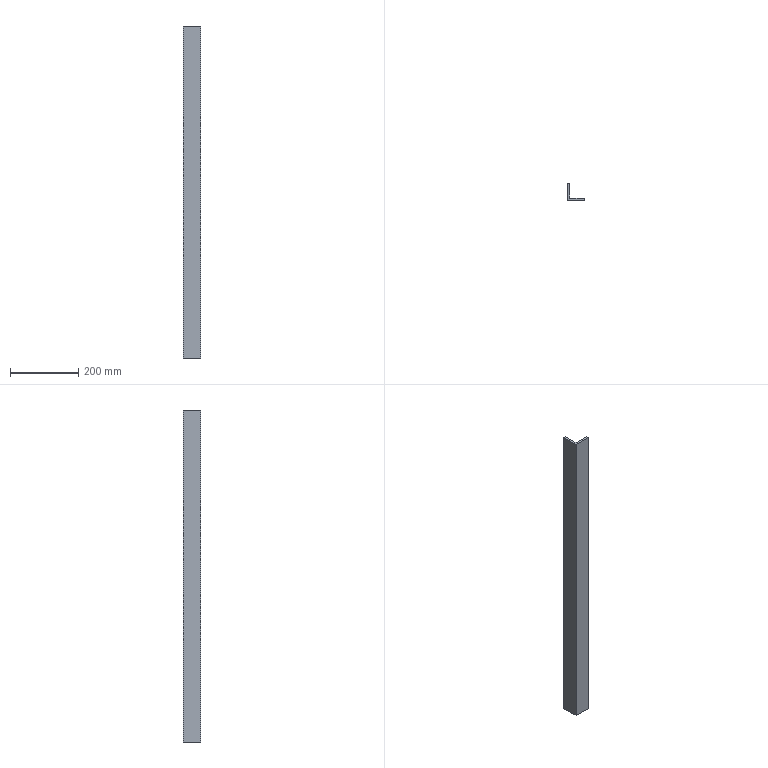Component | NX | VERTICAL_CORNER_PROTECTOR | 1 solid | 8 faces | box 50 x 50 x 975 mm | volume 549900 mm3 | plane 8
STEP:
#1=CARTESIAN_POINT('',(0.,0.,0.));
#2=DIRECTION('',(0.,0.,1.));
#3=DIRECTION('',(1.,0.,0.));
#4=AXIS2_PLACEMENT_3D('',#1,#2,#3);
#5=CARTESIAN_POINT('',(-622.5,-471.,0.));
#6=VERTEX_POINT('',#5);
#7=CARTESIAN_POINT('',(-628.5,-471.,0.));
#8=VERTEX_POINT('',#7);
#9=CARTESIAN_POINT('',(-622.5,-471.,0.));
#10=DIRECTION('',(-1.,0.,0.));
#11=VECTOR('',#10,1.);
#12=LINE('',#9,#11);
#13=CARTESIAN_POINT('',(-107.5,-60.,0.));
#14=DIRECTION('',(0.,0.,1.));
#15=DIRECTION('',(0.,-1.,0.));
#16=AXIS2_PLACEMENT_3D('',#13,#14,#15);
#17=PLANE('',#16);
#18=CARTESIAN_POINT('',(411.,-515.));
#19=DIRECTION('',(0.,-1.));
#20=VECTOR('',#19,1.);
#21=LINE('',#18,#20);
#22=(GEOMETRIC_REPRESENTATION_CONTEXT(2)PARAMETRIC_REPRESENTATION_CONTEXT()REPRESENTATION_CONTEXT('',''));
#23=DEFINITIONAL_REPRESENTATION('',(#21),#22);
#24=PCURVE('',#17,#23);
#25=CARTESIAN_POINT('',(-622.5,-471.,975.));
#26=DIRECTION('',(0.,-1.,0.));
#27=DIRECTION('',(0.,0.,-1.));
#28=AXIS2_PLACEMENT_3D('',#25,#26,#27);
#29=PLANE('',#28);
#30=CARTESIAN_POINT('',(975.,0.));
#31=DIRECTION('',(0.,-1.));
#32=VECTOR('',#31,1.);
#33=LINE('',#30,#32);
#34=(GEOMETRIC_REPRESENTATION_CONTEXT(2)PARAMETRIC_REPRESENTATION_CONTEXT()REPRESENTATION_CONTEXT('',''));
#35=DEFINITIONAL_REPRESENTATION('',(#33),#34);
#36=PCURVE('',#29,#35);
#37=SURFACE_CURVE('',#12,(#24,#36),.PCURVE_S1.);
#38=EDGE_CURVE('',#6,#8,#37,.T.);
#39=ORIENTED_EDGE('',*,*,#38,.F.);
#40=CARTESIAN_POINT('',(-622.5,-515.,0.));
#41=VERTEX_POINT('',#40);
#42=CARTESIAN_POINT('',(-622.5,730.,0.));
#43=DIRECTION('',(0.,-1.,0.));
#44=VECTOR('',#43,1.);
#45=LINE('',#42,#44);
#46=CARTESIAN_POINT('',(-790.,-515.));
#47=DIRECTION('',(1.,0.));
#48=VECTOR('',#47,1.);
#49=LINE('',#46,#48);
#50=(GEOMETRIC_REPRESENTATION_CONTEXT(2)PARAMETRIC_REPRESENTATION_CONTEXT()REPRESENTATION_CONTEXT('',''));
#51=DEFINITIONAL_REPRESENTATION('',(#49),#50);
#52=PCURVE('',#17,#51);
#53=CARTESIAN_POINT('',(-622.5,730.,975.));
#54=DIRECTION('',(1.,0.,0.));
#55=DIRECTION('',(0.,0.,1.));
#56=AXIS2_PLACEMENT_3D('',#53,#54,#55);
#57=PLANE('',#56);
#58=CARTESIAN_POINT('',(-975.,0.));
#59=DIRECTION('',(0.,1.));
#60=VECTOR('',#59,1.);
#61=LINE('',#58,#60);
#62=(GEOMETRIC_REPRESENTATION_CONTEXT(2)PARAMETRIC_REPRESENTATION_CONTEXT()REPRESENTATION_CONTEXT('',''));
#63=DEFINITIONAL_REPRESENTATION('',(#61),#62);
#64=PCURVE('',#57,#63);
#65=SURFACE_CURVE('',#45,(#52,#64),.PCURVE_S1.);
#66=EDGE_CURVE('',#6,#41,#65,.T.);
#67=ORIENTED_EDGE('',*,*,#66,.T.);
#68=CARTESIAN_POINT('',(-578.5,-515.,0.));
#69=VERTEX_POINT('',#68);
#70=CARTESIAN_POINT('',(-622.5,-515.,0.));
#71=DIRECTION('',(1.,0.,0.));
#72=VECTOR('',#71,1.);
#73=LINE('',#70,#72);
#74=CARTESIAN_POINT('',(455.,-515.));
#75=DIRECTION('',(0.,1.));
#76=VECTOR('',#75,1.);
#77=LINE('',#74,#76);
#78=(GEOMETRIC_REPRESENTATION_CONTEXT(2)PARAMETRIC_REPRESENTATION_CONTEXT()REPRESENTATION_CONTEXT('',''));
#79=DEFINITIONAL_REPRESENTATION('',(#77),#78);
#80=PCURVE('',#17,#79);
#81=CARTESIAN_POINT('',(-622.5,-515.,975.));
#82=DIRECTION('',(0.,1.,0.));
#83=DIRECTION('',(0.,0.,1.));
#84=AXIS2_PLACEMENT_3D('',#81,#82,#83);
#85=PLANE('',#84);
#86=CARTESIAN_POINT('',(-975.,0.));
#87=DIRECTION('',(0.,1.));
#88=VECTOR('',#87,1.);
#89=LINE('',#86,#88);
#90=(GEOMETRIC_REPRESENTATION_CONTEXT(2)PARAMETRIC_REPRESENTATION_CONTEXT()REPRESENTATION_CONTEXT('',''));
#91=DEFINITIONAL_REPRESENTATION('',(#89),#90);
#92=PCURVE('',#85,#91);
#93=SURFACE_CURVE('',#73,(#80,#92),.PCURVE_S1.);
#94=EDGE_CURVE('',#41,#69,#93,.T.);
#95=ORIENTED_EDGE('',*,*,#94,.T.);
#96=CARTESIAN_POINT('',(-578.5,-521.,0.));
#97=VERTEX_POINT('',#96);
#98=CARTESIAN_POINT('',(-578.5,-515.,0.));
#99=DIRECTION('',(0.,1.,0.));
#100=VECTOR('',#99,1.);
#101=LINE('',#98,#100);
#102=CARTESIAN_POINT('',(455.,-471.));
#103=DIRECTION('',(-1.,0.));
#104=VECTOR('',#103,1.);
#105=LINE('',#102,#104);
#106=(GEOMETRIC_REPRESENTATION_CONTEXT(2)PARAMETRIC_REPRESENTATION_CONTEXT()REPRESENTATION_CONTEXT('',''));
#107=DEFINITIONAL_REPRESENTATION('',(#105),#106);
#108=PCURVE('',#17,#107);
#109=CARTESIAN_POINT('',(-578.5,-515.,975.));
#110=DIRECTION('',(1.,0.,0.));
#111=DIRECTION('',(0.,0.,-1.));
#112=AXIS2_PLACEMENT_3D('',#109,#110,#111);
#113=PLANE('',#112);
#114=CARTESIAN_POINT('',(975.,0.));
#115=DIRECTION('',(0.,1.));
#116=VECTOR('',#115,1.);
#117=LINE('',#114,#116);
#118=(GEOMETRIC_REPRESENTATION_CONTEXT(2)PARAMETRIC_REPRESENTATION_CONTEXT()REPRESENTATION_CONTEXT('',''));
#119=DEFINITIONAL_REPRESENTATION('',(#117),#118);
#120=PCURVE('',#113,#119);
#121=SURFACE_CURVE('',#101,(#108,#120),.PCURVE_S1.);
#122=EDGE_CURVE('',#97,#69,#121,.T.);
#123=ORIENTED_EDGE('',*,*,#122,.F.);
#124=CARTESIAN_POINT('',(-628.5,-521.,0.));
#125=VERTEX_POINT('',#124);
#126=CARTESIAN_POINT('',(-622.5,-521.,0.));
#127=DIRECTION('',(1.,0.,0.));
#128=VECTOR('',#127,1.);
#129=LINE('',#126,#128);
#130=CARTESIAN_POINT('',(461.,-515.));
#131=DIRECTION('',(0.,1.));
#132=VECTOR('',#131,1.);
#133=LINE('',#130,#132);
#134=(GEOMETRIC_REPRESENTATION_CONTEXT(2)PARAMETRIC_REPRESENTATION_CONTEXT()REPRESENTATION_CONTEXT('',''));
#135=DEFINITIONAL_REPRESENTATION('',(#133),#134);
#136=PCURVE('',#17,#135);
#137=CARTESIAN_POINT('',(-622.5,-521.,975.));
#138=DIRECTION('',(0.,1.,0.));
#139=DIRECTION('',(0.,0.,1.));
#140=AXIS2_PLACEMENT_3D('',#137,#138,#139);
#141=PLANE('',#140);
#142=CARTESIAN_POINT('',(-975.,0.));
#143=DIRECTION('',(0.,1.));
#144=VECTOR('',#143,1.);
#145=LINE('',#142,#144);
#146=(GEOMETRIC_REPRESENTATION_CONTEXT(2)PARAMETRIC_REPRESENTATION_CONTEXT()REPRESENTATION_CONTEXT('',''));
#147=DEFINITIONAL_REPRESENTATION('',(#145),#146);
#148=PCURVE('',#141,#147);
#149=SURFACE_CURVE('',#129,(#136,#148),.PCURVE_S1.);
#150=EDGE_CURVE('',#125,#97,#149,.T.);
#151=ORIENTED_EDGE('',*,*,#150,.F.);
#152=CARTESIAN_POINT('',(-628.5,730.,0.));
#153=DIRECTION('',(0.,-1.,0.));
#154=VECTOR('',#153,1.);
#155=LINE('',#152,#154);
#156=CARTESIAN_POINT('',(-790.,-521.));
#157=DIRECTION('',(1.,0.));
#158=VECTOR('',#157,1.);
#159=LINE('',#156,#158);
#160=(GEOMETRIC_REPRESENTATION_CONTEXT(2)PARAMETRIC_REPRESENTATION_CONTEXT()REPRESENTATION_CONTEXT('',''));
#161=DEFINITIONAL_REPRESENTATION('',(#159),#160);
#162=PCURVE('',#17,#161);
#163=CARTESIAN_POINT('',(-628.5,730.,975.));
#164=DIRECTION('',(1.,0.,0.));
#165=DIRECTION('',(0.,0.,1.));
#166=AXIS2_PLACEMENT_3D('',#163,#164,#165);
#167=PLANE('',#166);
#168=CARTESIAN_POINT('',(-975.,0.));
#169=DIRECTION('',(0.,1.));
#170=VECTOR('',#169,1.);
#171=LINE('',#168,#170);
#172=(GEOMETRIC_REPRESENTATION_CONTEXT(2)PARAMETRIC_REPRESENTATION_CONTEXT()REPRESENTATION_CONTEXT('',''));
#173=DEFINITIONAL_REPRESENTATION('',(#171),#172);
#174=PCURVE('',#167,#173);
#175=SURFACE_CURVE('',#155,(#162,#174),.PCURVE_S1.);
#176=EDGE_CURVE('',#8,#125,#175,.T.);
#177=ORIENTED_EDGE('',*,*,#176,.F.);
#178=EDGE_LOOP('',(#39,#67,#95,#123,#151,#177));
#179=FACE_BOUND('',#178,.T.);
#180=ADVANCED_FACE('',(#179),#17,.F.);
#181=CARTESIAN_POINT('',(-622.5,-515.,975.));
#182=VERTEX_POINT('',#181);
#183=CARTESIAN_POINT('',(-578.5,-515.,975.));
#184=VERTEX_POINT('',#183);
#185=CARTESIAN_POINT('',(-622.5,-515.,975.));
#186=DIRECTION('',(1.,0.,0.));
#187=VECTOR('',#186,1.);
#188=LINE('',#185,#187);
#189=CARTESIAN_POINT('',(-622.5,-515.,975.));
#190=DIRECTION('',(0.,0.,1.));
#191=DIRECTION('',(1.,0.,0.));
#192=AXIS2_PLACEMENT_3D('',#189,#190,#191);
#193=PLANE('',#192);
#194=CARTESIAN_POINT('',(0.,0.));
#195=DIRECTION('',(1.,0.));
#196=VECTOR('',#195,1.);
#197=LINE('',#194,#196);
#198=(GEOMETRIC_REPRESENTATION_CONTEXT(2)PARAMETRIC_REPRESENTATION_CONTEXT()REPRESENTATION_CONTEXT('',''));
#199=DEFINITIONAL_REPRESENTATION('',(#197),#198);
#200=PCURVE('',#193,#199);
#201=CARTESIAN_POINT('',(0.,0.));
#202=DIRECTION('',(0.,1.));
#203=VECTOR('',#202,1.);
#204=LINE('',#201,#203);
#205=(GEOMETRIC_REPRESENTATION_CONTEXT(2)PARAMETRIC_REPRESENTATION_CONTEXT()REPRESENTATION_CONTEXT('',''));
#206=DEFINITIONAL_REPRESENTATION('',(#204),#205);
#207=PCURVE('',#85,#206);
#208=SURFACE_CURVE('',#188,(#200,#207),.PCURVE_S1.);
#209=EDGE_CURVE('',#182,#184,#208,.T.);
#210=ORIENTED_EDGE('',*,*,#209,.F.);
#211=CARTESIAN_POINT('',(-622.5,-471.,975.));
#212=VERTEX_POINT('',#211);
#213=CARTESIAN_POINT('',(-622.5,730.,975.));
#214=DIRECTION('',(0.,-1.,0.));
#215=VECTOR('',#214,1.);
#216=LINE('',#213,#215);
#217=CARTESIAN_POINT('',(0.,1245.));
#218=DIRECTION('',(0.,-1.));
#219=VECTOR('',#218,1.);
#220=LINE('',#217,#219);
#221=(GEOMETRIC_REPRESENTATION_CONTEXT(2)PARAMETRIC_REPRESENTATION_CONTEXT()REPRESENTATION_CONTEXT('',''));
#222=DEFINITIONAL_REPRESENTATION('',(#220),#221);
#223=PCURVE('',#193,#222);
#224=CARTESIAN_POINT('',(0.,0.));
#225=DIRECTION('',(0.,1.));
#226=VECTOR('',#225,1.);
#227=LINE('',#224,#226);
#228=(GEOMETRIC_REPRESENTATION_CONTEXT(2)PARAMETRIC_REPRESENTATION_CONTEXT()REPRESENTATION_CONTEXT('',''));
#229=DEFINITIONAL_REPRESENTATION('',(#227),#228);
#230=PCURVE('',#57,#229);
#231=SURFACE_CURVE('',#216,(#223,#230),.PCURVE_S1.);
#232=EDGE_CURVE('',#212,#182,#231,.T.);
#233=ORIENTED_EDGE('',*,*,#232,.F.);
#234=CARTESIAN_POINT('',(-628.5,-471.,975.));
#235=VERTEX_POINT('',#234);
#236=CARTESIAN_POINT('',(-622.5,-471.,975.));
#237=DIRECTION('',(-1.,0.,0.));
#238=VECTOR('',#237,1.);
#239=LINE('',#236,#238);
#240=CARTESIAN_POINT('',(0.,44.));
#241=DIRECTION('',(-1.,0.));
#242=VECTOR('',#241,1.);
#243=LINE('',#240,#242);
#244=(GEOMETRIC_REPRESENTATION_CONTEXT(2)PARAMETRIC_REPRESENTATION_CONTEXT()REPRESENTATION_CONTEXT('',''));
#245=DEFINITIONAL_REPRESENTATION('',(#243),#244);
#246=PCURVE('',#193,#245);
#247=CARTESIAN_POINT('',(0.,0.));
#248=DIRECTION('',(0.,-1.));
#249=VECTOR('',#248,1.);
#250=LINE('',#247,#249);
#251=(GEOMETRIC_REPRESENTATION_CONTEXT(2)PARAMETRIC_REPRESENTATION_CONTEXT()REPRESENTATION_CONTEXT('',''));
#252=DEFINITIONAL_REPRESENTATION('',(#250),#251);
#253=PCURVE('',#29,#252);
#254=SURFACE_CURVE('',#239,(#246,#253),.PCURVE_S1.);
#255=EDGE_CURVE('',#212,#235,#254,.T.);
#256=ORIENTED_EDGE('',*,*,#255,.T.);
#257=CARTESIAN_POINT('',(-628.5,-521.,975.));
#258=VERTEX_POINT('',#257);
#259=CARTESIAN_POINT('',(-628.5,730.,975.));
#260=DIRECTION('',(0.,-1.,0.));
#261=VECTOR('',#260,1.);
#262=LINE('',#259,#261);
#263=CARTESIAN_POINT('',(-6.,1245.));
#264=DIRECTION('',(0.,-1.));
#265=VECTOR('',#264,1.);
#266=LINE('',#263,#265);
#267=(GEOMETRIC_REPRESENTATION_CONTEXT(2)PARAMETRIC_REPRESENTATION_CONTEXT()REPRESENTATION_CONTEXT('',''));
#268=DEFINITIONAL_REPRESENTATION('',(#266),#267);
#269=PCURVE('',#193,#268);
#270=CARTESIAN_POINT('',(0.,0.));
#271=DIRECTION('',(0.,1.));
#272=VECTOR('',#271,1.);
#273=LINE('',#270,#272);
#274=(GEOMETRIC_REPRESENTATION_CONTEXT(2)PARAMETRIC_REPRESENTATION_CONTEXT()REPRESENTATION_CONTEXT('',''));
#275=DEFINITIONAL_REPRESENTATION('',(#273),#274);
#276=PCURVE('',#167,#275);
#277=SURFACE_CURVE('',#262,(#269,#276),.PCURVE_S1.);
#278=EDGE_CURVE('',#235,#258,#277,.T.);
#279=ORIENTED_EDGE('',*,*,#278,.T.);
#280=CARTESIAN_POINT('',(-578.5,-521.,975.));
#281=VERTEX_POINT('',#280);
#282=CARTESIAN_POINT('',(-622.5,-521.,975.));
#283=DIRECTION('',(1.,0.,0.));
#284=VECTOR('',#283,1.);
#285=LINE('',#282,#284);
#286=CARTESIAN_POINT('',(0.,-6.));
#287=DIRECTION('',(1.,0.));
#288=VECTOR('',#287,1.);
#289=LINE('',#286,#288);
#290=(GEOMETRIC_REPRESENTATION_CONTEXT(2)PARAMETRIC_REPRESENTATION_CONTEXT()REPRESENTATION_CONTEXT('',''));
#291=DEFINITIONAL_REPRESENTATION('',(#289),#290);
#292=PCURVE('',#193,#291);
#293=CARTESIAN_POINT('',(0.,0.));
#294=DIRECTION('',(0.,1.));
#295=VECTOR('',#294,1.);
#296=LINE('',#293,#295);
#297=(GEOMETRIC_REPRESENTATION_CONTEXT(2)PARAMETRIC_REPRESENTATION_CONTEXT()REPRESENTATION_CONTEXT('',''));
#298=DEFINITIONAL_REPRESENTATION('',(#296),#297);
#299=PCURVE('',#141,#298);
#300=SURFACE_CURVE('',#285,(#292,#299),.PCURVE_S1.);
#301=EDGE_CURVE('',#258,#281,#300,.T.);
#302=ORIENTED_EDGE('',*,*,#301,.T.);
#303=CARTESIAN_POINT('',(-578.5,-515.,975.));
#304=DIRECTION('',(0.,-1.,0.));
#305=VECTOR('',#304,1.);
#306=LINE('',#303,#305);
#307=CARTESIAN_POINT('',(44.,0.));
#308=DIRECTION('',(0.,-1.));
#309=VECTOR('',#308,1.);
#310=LINE('',#307,#309);
#311=(GEOMETRIC_REPRESENTATION_CONTEXT(2)PARAMETRIC_REPRESENTATION_CONTEXT()REPRESENTATION_CONTEXT('',''));
#312=DEFINITIONAL_REPRESENTATION('',(#310),#311);
#313=PCURVE('',#193,#312);
#314=CARTESIAN_POINT('',(0.,0.));
#315=DIRECTION('',(0.,-1.));
#316=VECTOR('',#315,1.);
#317=LINE('',#314,#316);
#318=(GEOMETRIC_REPRESENTATION_CONTEXT(2)PARAMETRIC_REPRESENTATION_CONTEXT()REPRESENTATION_CONTEXT('',''));
#319=DEFINITIONAL_REPRESENTATION('',(#317),#318);
#320=PCURVE('',#113,#319);
#321=SURFACE_CURVE('',#306,(#313,#320),.PCURVE_S1.);
#322=EDGE_CURVE('',#184,#281,#321,.T.);
#323=ORIENTED_EDGE('',*,*,#322,.F.);
#324=EDGE_LOOP('',(#210,#233,#256,#279,#302,#323));
#325=FACE_BOUND('',#324,.T.);
#326=ADVANCED_FACE('',(#325),#193,.T.);
#327=CARTESIAN_POINT('',(-578.5,-521.,975.));
#328=DIRECTION('',(0.,0.,-1.));
#329=VECTOR('',#328,1.);
#330=LINE('',#327,#329);
#331=CARTESIAN_POINT('',(0.,-6.));
#332=DIRECTION('',(1.,0.));
#333=VECTOR('',#332,1.);
#334=LINE('',#331,#333);
#335=(GEOMETRIC_REPRESENTATION_CONTEXT(2)PARAMETRIC_REPRESENTATION_CONTEXT()REPRESENTATION_CONTEXT('',''));
#336=DEFINITIONAL_REPRESENTATION('',(#334),#335);
#337=PCURVE('',#113,#336);
#338=CARTESIAN_POINT('',(0.,44.));
#339=DIRECTION('',(-1.,0.));
#340=VECTOR('',#339,1.);
#341=LINE('',#338,#340);
#342=(GEOMETRIC_REPRESENTATION_CONTEXT(2)PARAMETRIC_REPRESENTATION_CONTEXT()REPRESENTATION_CONTEXT('',''));
#343=DEFINITIONAL_REPRESENTATION('',(#341),#342);
#344=PCURVE('',#141,#343);
#345=SURFACE_CURVE('',#330,(#337,#344),.PCURVE_S1.);
#346=EDGE_CURVE('',#281,#97,#345,.T.);
#347=ORIENTED_EDGE('',*,*,#346,.T.);
#348=ORIENTED_EDGE('',*,*,#122,.T.);
#349=CARTESIAN_POINT('',(-578.5,-515.,975.));
#350=DIRECTION('',(0.,0.,-1.));
#351=VECTOR('',#350,1.);
#352=LINE('',#349,#351);
#353=CARTESIAN_POINT('',(0.,0.));
#354=DIRECTION('',(1.,0.));
#355=VECTOR('',#354,1.);
#356=LINE('',#353,#355);
#357=(GEOMETRIC_REPRESENTATION_CONTEXT(2)PARAMETRIC_REPRESENTATION_CONTEXT()REPRESENTATION_CONTEXT('',''));
#358=DEFINITIONAL_REPRESENTATION('',(#356),#357);
#359=PCURVE('',#113,#358);
#360=CARTESIAN_POINT('',(0.,44.));
#361=DIRECTION('',(-1.,0.));
#362=VECTOR('',#361,1.);
#363=LINE('',#360,#362);
#364=(GEOMETRIC_REPRESENTATION_CONTEXT(2)PARAMETRIC_REPRESENTATION_CONTEXT()REPRESENTATION_CONTEXT('',''));
#365=DEFINITIONAL_REPRESENTATION('',(#363),#364);
#366=PCURVE('',#85,#365);
#367=SURFACE_CURVE('',#352,(#359,#366),.PCURVE_S1.);
#368=EDGE_CURVE('',#184,#69,#367,.T.);
#369=ORIENTED_EDGE('',*,*,#368,.F.);
#370=ORIENTED_EDGE('',*,*,#322,.T.);
#371=EDGE_LOOP('',(#347,#348,#369,#370));
#372=FACE_BOUND('',#371,.T.);
#373=ADVANCED_FACE('',(#372),#113,.T.);
#374=CARTESIAN_POINT('',(-622.5,-471.,975.));
#375=DIRECTION('',(0.,0.,-1.));
#376=VECTOR('',#375,1.);
#377=LINE('',#374,#376);
#378=CARTESIAN_POINT('',(0.,0.));
#379=DIRECTION('',(1.,0.));
#380=VECTOR('',#379,1.);
#381=LINE('',#378,#380);
#382=(GEOMETRIC_REPRESENTATION_CONTEXT(2)PARAMETRIC_REPRESENTATION_CONTEXT()REPRESENTATION_CONTEXT('',''));
#383=DEFINITIONAL_REPRESENTATION('',(#381),#382);
#384=PCURVE('',#29,#383);
#385=CARTESIAN_POINT('',(0.,1201.));
#386=DIRECTION('',(-1.,0.));
#387=VECTOR('',#386,1.);
#388=LINE('',#385,#387);
#389=(GEOMETRIC_REPRESENTATION_CONTEXT(2)PARAMETRIC_REPRESENTATION_CONTEXT()REPRESENTATION_CONTEXT('',''));
#390=DEFINITIONAL_REPRESENTATION('',(#388),#389);
#391=PCURVE('',#57,#390);
#392=SURFACE_CURVE('',#377,(#384,#391),.PCURVE_S1.);
#393=EDGE_CURVE('',#212,#6,#392,.T.);
#394=ORIENTED_EDGE('',*,*,#393,.T.);
#395=ORIENTED_EDGE('',*,*,#38,.T.);
#396=CARTESIAN_POINT('',(-628.5,-471.,975.));
#397=DIRECTION('',(0.,0.,-1.));
#398=VECTOR('',#397,1.);
#399=LINE('',#396,#398);
#400=CARTESIAN_POINT('',(0.,-6.));
#401=DIRECTION('',(1.,0.));
#402=VECTOR('',#401,1.);
#403=LINE('',#400,#402);
#404=(GEOMETRIC_REPRESENTATION_CONTEXT(2)PARAMETRIC_REPRESENTATION_CONTEXT()REPRESENTATION_CONTEXT('',''));
#405=DEFINITIONAL_REPRESENTATION('',(#403),#404);
#406=PCURVE('',#29,#405);
#407=CARTESIAN_POINT('',(0.,1201.));
#408=DIRECTION('',(-1.,0.));
#409=VECTOR('',#408,1.);
#410=LINE('',#407,#409);
#411=(GEOMETRIC_REPRESENTATION_CONTEXT(2)PARAMETRIC_REPRESENTATION_CONTEXT()REPRESENTATION_CONTEXT('',''));
#412=DEFINITIONAL_REPRESENTATION('',(#410),#411);
#413=PCURVE('',#167,#412);
#414=SURFACE_CURVE('',#399,(#406,#413),.PCURVE_S1.);
#415=EDGE_CURVE('',#235,#8,#414,.T.);
#416=ORIENTED_EDGE('',*,*,#415,.F.);
#417=ORIENTED_EDGE('',*,*,#255,.F.);
#418=EDGE_LOOP('',(#394,#395,#416,#417));
#419=FACE_BOUND('',#418,.T.);
#420=ADVANCED_FACE('',(#419),#29,.F.);
#421=ORIENTED_EDGE('',*,*,#415,.T.);
#422=ORIENTED_EDGE('',*,*,#176,.T.);
#423=CARTESIAN_POINT('',(-628.5,-521.,975.));
#424=DIRECTION('',(0.,0.,-1.));
#425=VECTOR('',#424,1.);
#426=LINE('',#423,#425);
#427=CARTESIAN_POINT('',(0.,1251.));
#428=DIRECTION('',(-1.,0.));
#429=VECTOR('',#428,1.);
#430=LINE('',#427,#429);
#431=(GEOMETRIC_REPRESENTATION_CONTEXT(2)PARAMETRIC_REPRESENTATION_CONTEXT()REPRESENTATION_CONTEXT('',''));
#432=DEFINITIONAL_REPRESENTATION('',(#430),#431);
#433=PCURVE('',#167,#432);
#434=CARTESIAN_POINT('',(0.,-6.));
#435=DIRECTION('',(-1.,0.));
#436=VECTOR('',#435,1.);
#437=LINE('',#434,#436);
#438=(GEOMETRIC_REPRESENTATION_CONTEXT(2)PARAMETRIC_REPRESENTATION_CONTEXT()REPRESENTATION_CONTEXT('',''));
#439=DEFINITIONAL_REPRESENTATION('',(#437),#438);
#440=PCURVE('',#141,#439);
#441=SURFACE_CURVE('',#426,(#433,#440),.PCURVE_S1.);
#442=EDGE_CURVE('',#258,#125,#441,.T.);
#443=ORIENTED_EDGE('',*,*,#442,.F.);
#444=ORIENTED_EDGE('',*,*,#278,.F.);
#445=EDGE_LOOP('',(#421,#422,#443,#444));
#446=FACE_BOUND('',#445,.T.);
#447=ADVANCED_FACE('',(#446),#167,.F.);
#448=ORIENTED_EDGE('',*,*,#442,.T.);
#449=ORIENTED_EDGE('',*,*,#150,.T.);
#450=ORIENTED_EDGE('',*,*,#346,.F.);
#451=ORIENTED_EDGE('',*,*,#301,.F.);
#452=EDGE_LOOP('',(#448,#449,#450,#451));
#453=FACE_BOUND('',#452,.T.);
#454=ADVANCED_FACE('',(#453),#141,.F.);
#455=ORIENTED_EDGE('',*,*,#66,.F.);
#456=ORIENTED_EDGE('',*,*,#393,.F.);
#457=ORIENTED_EDGE('',*,*,#232,.T.);
#458=CARTESIAN_POINT('',(-622.5,-515.,975.));
#459=DIRECTION('',(0.,0.,-1.));
#460=VECTOR('',#459,1.);
#461=LINE('',#458,#460);
#462=CARTESIAN_POINT('',(0.,1245.));
#463=DIRECTION('',(-1.,0.));
#464=VECTOR('',#463,1.);
#465=LINE('',#462,#464);
#466=(GEOMETRIC_REPRESENTATION_CONTEXT(2)PARAMETRIC_REPRESENTATION_CONTEXT()REPRESENTATION_CONTEXT('',''));
#467=DEFINITIONAL_REPRESENTATION('',(#465),#466);
#468=PCURVE('',#57,#467);
#469=CARTESIAN_POINT('',(0.,0.));
#470=DIRECTION('',(-1.,0.));
#471=VECTOR('',#470,1.);
#472=LINE('',#469,#471);
#473=(GEOMETRIC_REPRESENTATION_CONTEXT(2)PARAMETRIC_REPRESENTATION_CONTEXT()REPRESENTATION_CONTEXT('',''));
#474=DEFINITIONAL_REPRESENTATION('',(#472),#473);
#475=PCURVE('',#85,#474);
#476=SURFACE_CURVE('',#461,(#468,#475),.PCURVE_S1.);
#477=EDGE_CURVE('',#182,#41,#476,.T.);
#478=ORIENTED_EDGE('',*,*,#477,.T.);
#479=EDGE_LOOP('',(#455,#456,#457,#478));
#480=FACE_BOUND('',#479,.T.);
#481=ADVANCED_FACE('',(#480),#57,.T.);
#482=ORIENTED_EDGE('',*,*,#94,.F.);
#483=ORIENTED_EDGE('',*,*,#477,.F.);
#484=ORIENTED_EDGE('',*,*,#209,.T.);
#485=ORIENTED_EDGE('',*,*,#368,.T.);
#486=EDGE_LOOP('',(#482,#483,#484,#485));
#487=FACE_BOUND('',#486,.T.);
#488=ADVANCED_FACE('',(#487),#85,.T.);
#489=CLOSED_SHELL('',(#180,#326,#373,#420,#447,#454,#481,#488));
#490=MANIFOLD_SOLID_BREP('',#489);
#491=(LENGTH_UNIT()NAMED_UNIT(*)SI_UNIT(.MILLI.,.METRE.));
#492=UNCERTAINTY_MEASURE_WITH_UNIT(LENGTH_MEASURE(0.0000001),#491,'','');
#493=(NAMED_UNIT(*)PLANE_ANGLE_UNIT()SI_UNIT($,.RADIAN.));
#494=(NAMED_UNIT(*)SI_UNIT($,.STERADIAN.)SOLID_ANGLE_UNIT());
#495=(GEOMETRIC_REPRESENTATION_CONTEXT(3)GLOBAL_UNCERTAINTY_ASSIGNED_CONTEXT((#492))GLOBAL_UNIT_ASSIGNED_CONTEXT((#491,#493,#494))REPRESENTATION_CONTEXT('',''));
#496=ADVANCED_BREP_SHAPE_REPRESENTATION('',(#4,#490),#495);